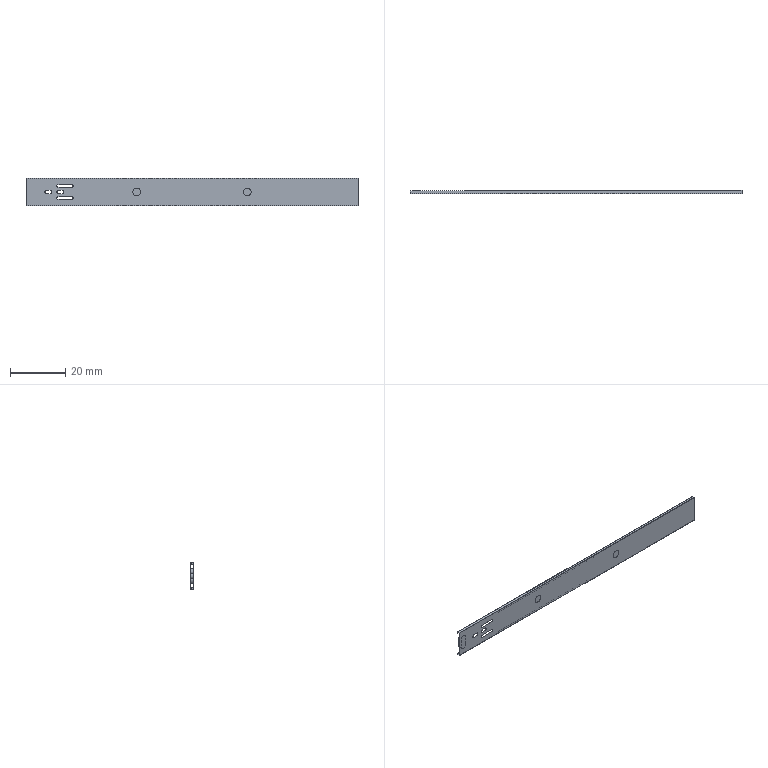Component | NX | SLIDE_RAIL_SMALL | 2 solids | 79 faces | volume 275 mm3 | plane 53 | cylinder 26 | commonest cylinder face diameters 1.5 x10 2.5 x4 1.2 x4 1 x4 2.8 x2 3 x2